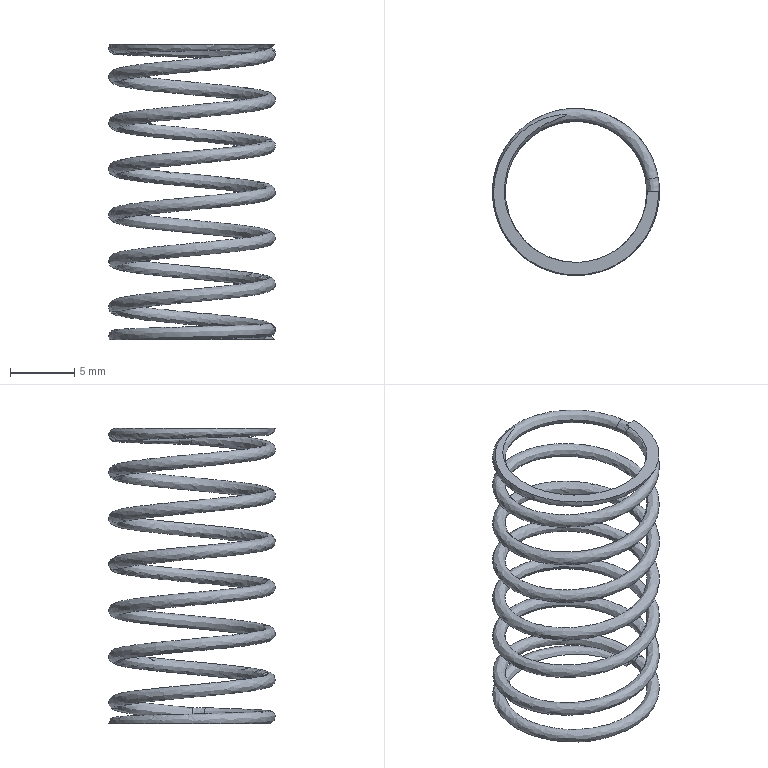Component | NX | SPRING_2 | 1 solid | 9 faces | volume 216 mm3 | spline 5 | plane 4